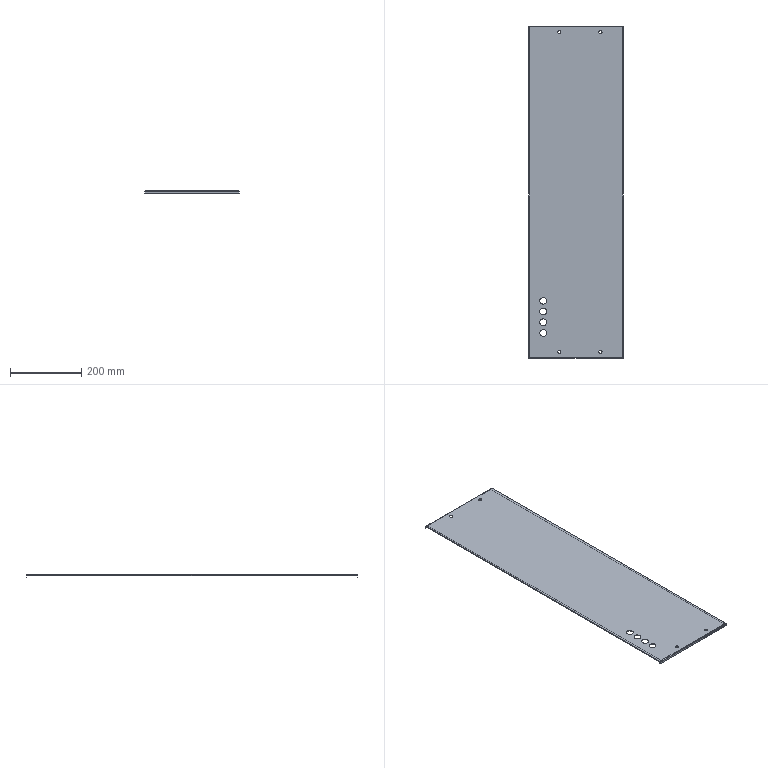Component | SolidWorks | FrontSealingPlate100-1 | 1 solid | 58 faces | volume 309127 mm3 | plane 34 | cylinder 24 | commonest cylinder face diameters 9 x8 19 x8 4.8 x2 2.4 x2 2.5 x2 0.1 x2